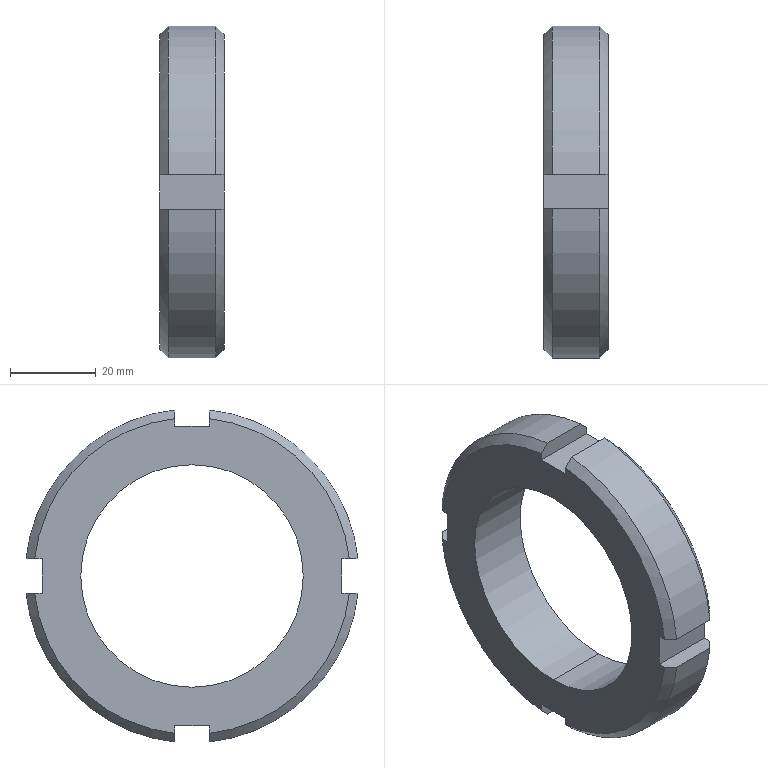Component | SolidWorks | 4RoundNutM52X1.5-1 | 1 solid | 28 faces | box 15 x 77.59 x 77.59 mm | volume 37097 mm3 | plane 14 | cone 8 | cylinder 6 | commonest cylinder face diameters 78 x4 52 x2
build123d program:
from build123d import *

# Parameters (mm, degrees)
SKETCH1_R              = 39
BOSS_EXTRUDE1_DEPTH    = 15
M52X5_0_TAPPED_HOLE1_D = 52
SKETCH5_W              = 8
SKETCH5_H              = 8
CUT_EXTRUDE1_DEPTH     = 15
CIRPATTERN1_COUNT      = 4
CHAMFER1_SIZE          = 2


with BuildPart() as part:
    # Sketch1 → Boss-Extrude1 (new body)
    with BuildSketch(Plane.XY):
        Circle(SKETCH1_R)
    extrude(amount=BOSS_EXTRUDE1_DEPTH)

    # M52x5.0 Tapped Hole1 (through all)
    with Locations(Plane.XY.offset(15)):
        with Locations((0, 0)):
            Hole(M52X5_0_TAPPED_HOLE1_D / 2)

    # Sketch5 → Cut-Extrude1 (cut)
    with BuildSketch(Plane.XY.offset(15)):
        with Locations((0, 39)):
            Rectangle(SKETCH5_W, SKETCH5_H)
    cut_extrude1 = extrude(amount=-CUT_EXTRUDE1_DEPTH, mode=Mode.SUBTRACT)

    # CirPattern1: Cut-Extrude1 ×4 about axis
    cirpattern1_axis = Axis((0, 0, 0), (0, 0, 1))
    for i in range(1, CIRPATTERN1_COUNT):
        add(cut_extrude1.rotate(cirpattern1_axis, i * 360 / CIRPATTERN1_COUNT), mode=Mode.SUBTRACT)

    # Chamfer1
    chamfer1_edges = [part.edges().sort_by_distance(p)[0] for p in [
        (-27.577, 27.577, 0),
        (-27.577, 27.577, 15),
        (27.577, 27.577, 0),
        (27.577, 27.577, 15),
        (-27.577, -27.577, 0),
        (27.577, -27.577, 0),
        (-27.577, -27.577, 15),
        (27.577, -27.577, 15),
    ]]
    chamfer(chamfer1_edges, length=CHAMFER1_SIZE)


solid = part.part

# Placed as in the assembly
solid = solid.moved(Location((72.957, 1.776, 250), (0, 90, 0)))
STEP:
#1=COLOUR_RGB('',0.7922,0.8196,0.9333);
#2=FILL_AREA_STYLE_COLOUR('',#1);
#3=FILL_AREA_STYLE('',(#2));
#4=SURFACE_STYLE_FILL_AREA(#3);
#5=SURFACE_SIDE_STYLE('',(#4));
#6=SURFACE_STYLE_USAGE(.BOTH.,#5);
#7=PRESENTATION_STYLE_ASSIGNMENT((#6));
#8=CARTESIAN_POINT('',(3.463,0.06992,8.819));
#9=VERTEX_POINT('',#8);
#10=CARTESIAN_POINT('',(3.463,0.06992,10.866));
#11=VERTEX_POINT('',#10);
#12=CARTESIAN_POINT('',(3.463,0.06992,9.843));
#13=DIRECTION('',(-1.,-0.,-0.));
#14=DIRECTION('',(0.,0.,1.));
#15=AXIS2_PLACEMENT_3D('',#12,#13,#14);
#16=CIRCLE('',#15,1.024);
#17=EDGE_CURVE('',#9,#11,#16,.T.);
#18=ORIENTED_EDGE('',*,*,#17,.F.);
#19=CARTESIAN_POINT('',(2.872,0.06992,8.819));
#20=VERTEX_POINT('',#19);
#21=CARTESIAN_POINT('',(2.872,0.06992,8.819));
#22=DIRECTION('',(-1.,-0.,-0.));
#23=VECTOR('',#22,39.37);
#24=LINE('',#21,#23);
#25=EDGE_CURVE('',#9,#20,#24,.T.);
#26=ORIENTED_EDGE('',*,*,#25,.T.);
#27=CARTESIAN_POINT('',(2.872,0.06992,10.866));
#28=VERTEX_POINT('',#27);
#29=CARTESIAN_POINT('',(2.872,0.06992,9.843));
#30=DIRECTION('',(-1.,-0.,-0.));
#31=DIRECTION('',(0.,0.,1.));
#32=AXIS2_PLACEMENT_3D('',#29,#30,#31);
#33=CIRCLE('',#32,1.024);
#34=EDGE_CURVE('',#20,#28,#33,.T.);
#35=ORIENTED_EDGE('',*,*,#34,.T.);
#36=CARTESIAN_POINT('',(2.872,0.06992,10.866));
#37=DIRECTION('',(-1.,-0.,-0.));
#38=VECTOR('',#37,39.37);
#39=LINE('',#36,#38);
#40=EDGE_CURVE('',#11,#28,#39,.T.);
#41=ORIENTED_EDGE('',*,*,#40,.F.);
#42=EDGE_LOOP('',(#18,#26,#35,#41));
#43=FACE_OUTER_BOUND('',#42,.T.);
#44=CARTESIAN_POINT('',(2.872,0.06992,9.843));
#45=DIRECTION('',(-1.,-0.,-0.));
#46=DIRECTION('',(0.,0.,1.));
#47=AXIS2_PLACEMENT_3D('',#44,#45,#46);
#48=CYLINDRICAL_SURFACE('',#47,1.024);
#49=ADVANCED_FACE('',(#43),#48,.F.);
#50=CARTESIAN_POINT('',(2.951,-0.08756,8.315));
#51=VERTEX_POINT('',#50);
#52=CARTESIAN_POINT('',(3.384,-0.08756,8.315));
#53=VERTEX_POINT('',#52);
#54=CARTESIAN_POINT('',(2.872,-0.08756,8.315));
#55=DIRECTION('',(1.,0.,0.));
#56=VECTOR('',#55,39.37);
#57=LINE('',#54,#56);
#58=EDGE_CURVE('',#51,#53,#57,.T.);
#59=ORIENTED_EDGE('',*,*,#58,.T.);
#60=CARTESIAN_POINT('',(3.384,-1.457,9.685));
#61=VERTEX_POINT('',#60);
#62=CARTESIAN_POINT('',(3.384,0.06992,9.843));
#63=DIRECTION('',(-1.,-0.,-0.));
#64=DIRECTION('',(0.,-0.,1.));
#65=AXIS2_PLACEMENT_3D('',#62,#63,#64);
#66=CIRCLE('',#65,1.535);
#67=EDGE_CURVE('',#53,#61,#66,.T.);
#68=ORIENTED_EDGE('',*,*,#67,.T.);
#69=CARTESIAN_POINT('',(2.951,-1.457,9.685));
#70=VERTEX_POINT('',#69);
#71=CARTESIAN_POINT('',(2.872,-1.457,9.685));
#72=DIRECTION('',(-1.,-0.,-0.));
#73=VECTOR('',#72,39.37);
#74=LINE('',#71,#73);
#75=EDGE_CURVE('',#61,#70,#74,.T.);
#76=ORIENTED_EDGE('',*,*,#75,.T.);
#77=CARTESIAN_POINT('',(2.951,0.06992,9.843));
#78=DIRECTION('',(1.,0.,0.));
#79=DIRECTION('',(0.,-0.,1.));
#80=AXIS2_PLACEMENT_3D('',#77,#78,#79);
#81=CIRCLE('',#80,1.535);
#82=EDGE_CURVE('',#70,#51,#81,.T.);
#83=ORIENTED_EDGE('',*,*,#82,.T.);
#84=EDGE_LOOP('',(#59,#68,#76,#83));
#85=FACE_OUTER_BOUND('',#84,.T.);
#86=CARTESIAN_POINT('',(2.872,0.06992,9.843));
#87=DIRECTION('',(1.,0.,0.));
#88=DIRECTION('',(0.,0.,-1.));
#89=AXIS2_PLACEMENT_3D('',#86,#87,#88);
#90=CYLINDRICAL_SURFACE('',#89,1.535);
#91=ADVANCED_FACE('',(#85),#90,.T.);
#92=CARTESIAN_POINT('',(2.951,1.597,9.685));
#93=VERTEX_POINT('',#92);
#94=CARTESIAN_POINT('',(3.384,1.597,9.685));
#95=VERTEX_POINT('',#94);
#96=CARTESIAN_POINT('',(2.872,1.597,9.685));
#97=DIRECTION('',(1.,0.,0.));
#98=VECTOR('',#97,39.37);
#99=LINE('',#96,#98);
#100=EDGE_CURVE('',#93,#95,#99,.T.);
#101=ORIENTED_EDGE('',*,*,#100,.T.);
#102=CARTESIAN_POINT('',(3.384,0.2274,8.315));
#103=VERTEX_POINT('',#102);
#104=CARTESIAN_POINT('',(3.384,0.06992,9.843));
#105=DIRECTION('',(-1.,-0.,-0.));
#106=DIRECTION('',(0.,-0.,1.));
#107=AXIS2_PLACEMENT_3D('',#104,#105,#106);
#108=CIRCLE('',#107,1.535);
#109=EDGE_CURVE('',#95,#103,#108,.T.);
#110=ORIENTED_EDGE('',*,*,#109,.T.);
#111=CARTESIAN_POINT('',(2.951,0.2274,8.315));
#112=VERTEX_POINT('',#111);
#113=CARTESIAN_POINT('',(2.872,0.2274,8.315));
#114=DIRECTION('',(-1.,-0.,-0.));
#115=VECTOR('',#114,39.37);
#116=LINE('',#113,#115);
#117=EDGE_CURVE('',#103,#112,#116,.T.);
#118=ORIENTED_EDGE('',*,*,#117,.T.);
#119=CARTESIAN_POINT('',(2.951,0.06992,9.843));
#120=DIRECTION('',(1.,0.,0.));
#121=DIRECTION('',(0.,-0.,1.));
#122=AXIS2_PLACEMENT_3D('',#119,#120,#121);
#123=CIRCLE('',#122,1.535);
#124=EDGE_CURVE('',#112,#93,#123,.T.);
#125=ORIENTED_EDGE('',*,*,#124,.T.);
#126=EDGE_LOOP('',(#101,#110,#118,#125));
#127=FACE_OUTER_BOUND('',#126,.T.);
#128=CARTESIAN_POINT('',(2.872,0.06992,9.843));
#129=DIRECTION('',(1.,0.,0.));
#130=DIRECTION('',(0.,0.,-1.));
#131=AXIS2_PLACEMENT_3D('',#128,#129,#130);
#132=CYLINDRICAL_SURFACE('',#131,1.535);
#133=ADVANCED_FACE('',(#127),#132,.T.);
#134=CARTESIAN_POINT('',(2.951,-1.457,10.));
#135=VERTEX_POINT('',#134);
#136=CARTESIAN_POINT('',(3.384,-1.457,10.));
#137=VERTEX_POINT('',#136);
#138=CARTESIAN_POINT('',(2.872,-1.457,10.));
#139=DIRECTION('',(1.,0.,0.));
#140=VECTOR('',#139,39.37);
#141=LINE('',#138,#140);
#142=EDGE_CURVE('',#135,#137,#141,.T.);
#143=ORIENTED_EDGE('',*,*,#142,.T.);
#144=CARTESIAN_POINT('',(3.384,-0.08756,11.37));
#145=VERTEX_POINT('',#144);
#146=CARTESIAN_POINT('',(3.384,0.06992,9.843));
#147=DIRECTION('',(-1.,-0.,-0.));
#148=DIRECTION('',(0.,-0.,1.));
#149=AXIS2_PLACEMENT_3D('',#146,#147,#148);
#150=CIRCLE('',#149,1.535);
#151=EDGE_CURVE('',#137,#145,#150,.T.);
#152=ORIENTED_EDGE('',*,*,#151,.T.);
#153=CARTESIAN_POINT('',(2.951,-0.08756,11.37));
#154=VERTEX_POINT('',#153);
#155=CARTESIAN_POINT('',(2.872,-0.08756,11.37));
#156=DIRECTION('',(-1.,-0.,-0.));
#157=VECTOR('',#156,39.37);
#158=LINE('',#155,#157);
#159=EDGE_CURVE('',#145,#154,#158,.T.);
#160=ORIENTED_EDGE('',*,*,#159,.T.);
#161=CARTESIAN_POINT('',(2.951,0.06992,9.843));
#162=DIRECTION('',(1.,0.,0.));
#163=DIRECTION('',(0.,-0.,1.));
#164=AXIS2_PLACEMENT_3D('',#161,#162,#163);
#165=CIRCLE('',#164,1.535);
#166=EDGE_CURVE('',#154,#135,#165,.T.);
#167=ORIENTED_EDGE('',*,*,#166,.T.);
#168=EDGE_LOOP('',(#143,#152,#160,#167));
#169=FACE_OUTER_BOUND('',#168,.T.);
#170=CARTESIAN_POINT('',(2.872,0.06992,9.843));
#171=DIRECTION('',(1.,0.,0.));
#172=DIRECTION('',(0.,0.,-1.));
#173=AXIS2_PLACEMENT_3D('',#170,#171,#172);
#174=CYLINDRICAL_SURFACE('',#173,1.535);
#175=ADVANCED_FACE('',(#169),#174,.T.);
#176=CARTESIAN_POINT('',(2.951,0.2274,11.37));
#177=VERTEX_POINT('',#176);
#178=CARTESIAN_POINT('',(3.384,0.2274,11.37));
#179=VERTEX_POINT('',#178);
#180=CARTESIAN_POINT('',(2.872,0.2274,11.37));
#181=DIRECTION('',(1.,0.,0.));
#182=VECTOR('',#181,39.37);
#183=LINE('',#180,#182);
#184=EDGE_CURVE('',#177,#179,#183,.T.);
#185=ORIENTED_EDGE('',*,*,#184,.T.);
#186=CARTESIAN_POINT('',(3.384,1.597,10.));
#187=VERTEX_POINT('',#186);
#188=CARTESIAN_POINT('',(3.384,0.06992,9.843));
#189=DIRECTION('',(-1.,-0.,-0.));
#190=DIRECTION('',(0.,-0.,1.));
#191=AXIS2_PLACEMENT_3D('',#188,#189,#190);
#192=CIRCLE('',#191,1.535);
#193=EDGE_CURVE('',#179,#187,#192,.T.);
#194=ORIENTED_EDGE('',*,*,#193,.T.);
#195=CARTESIAN_POINT('',(2.951,1.597,10.));
#196=VERTEX_POINT('',#195);
#197=CARTESIAN_POINT('',(2.872,1.597,10.));
#198=DIRECTION('',(-1.,-0.,-0.));
#199=VECTOR('',#198,39.37);
#200=LINE('',#197,#199);
#201=EDGE_CURVE('',#187,#196,#200,.T.);
#202=ORIENTED_EDGE('',*,*,#201,.T.);
#203=CARTESIAN_POINT('',(2.951,0.06992,9.843));
#204=DIRECTION('',(1.,0.,0.));
#205=DIRECTION('',(0.,-0.,1.));
#206=AXIS2_PLACEMENT_3D('',#203,#204,#205);
#207=CIRCLE('',#206,1.535);
#208=EDGE_CURVE('',#196,#177,#207,.T.);
#209=ORIENTED_EDGE('',*,*,#208,.T.);
#210=EDGE_LOOP('',(#185,#194,#202,#209));
#211=FACE_OUTER_BOUND('',#210,.T.);
#212=CARTESIAN_POINT('',(2.872,0.06992,9.843));
#213=DIRECTION('',(1.,0.,0.));
#214=DIRECTION('',(0.,0.,-1.));
#215=AXIS2_PLACEMENT_3D('',#212,#213,#214);
#216=CYLINDRICAL_SURFACE('',#215,1.535);
#217=ADVANCED_FACE('',(#211),#216,.T.);
#218=CARTESIAN_POINT('',(2.872,-1.378,10.));
#219=VERTEX_POINT('',#218);
#220=CARTESIAN_POINT('',(2.872,-1.308,10.));
#221=VERTEX_POINT('',#220);
#222=CARTESIAN_POINT('',(2.872,-1.308,10.));
#223=DIRECTION('',(-0.,1.,0.));
#224=VECTOR('',#223,39.37);
#225=LINE('',#222,#224);
#226=EDGE_CURVE('',#219,#221,#225,.T.);
#227=ORIENTED_EDGE('',*,*,#226,.F.);
#228=CARTESIAN_POINT('',(2.872,-0.08756,11.291));
#229=VERTEX_POINT('',#228);
#230=CARTESIAN_POINT('',(2.872,0.06992,9.843));
#231=DIRECTION('',(-1.,-0.,-0.));
#232=DIRECTION('',(0.,-0.,1.));
#233=AXIS2_PLACEMENT_3D('',#230,#231,#232);
#234=CIRCLE('',#233,1.457);
#235=EDGE_CURVE('',#219,#229,#234,.T.);
#236=ORIENTED_EDGE('',*,*,#235,.T.);
#237=CARTESIAN_POINT('',(2.872,-0.08756,11.22));
#238=VERTEX_POINT('',#237);
#239=CARTESIAN_POINT('',(2.872,-0.08756,11.22));
#240=DIRECTION('',(-0.,-0.,1.));
#241=VECTOR('',#240,39.37);
#242=LINE('',#239,#241);
#243=EDGE_CURVE('',#238,#229,#242,.T.);
#244=ORIENTED_EDGE('',*,*,#243,.F.);
#245=CARTESIAN_POINT('',(2.872,0.2274,11.22));
#246=VERTEX_POINT('',#245);
#247=CARTESIAN_POINT('',(2.872,0.2274,11.22));
#248=DIRECTION('',(0.,-1.,-0.));
#249=VECTOR('',#248,39.37);
#250=LINE('',#247,#249);
#251=EDGE_CURVE('',#246,#238,#250,.T.);
#252=ORIENTED_EDGE('',*,*,#251,.F.);
#253=CARTESIAN_POINT('',(2.872,0.2274,11.291));
#254=VERTEX_POINT('',#253);
#255=CARTESIAN_POINT('',(2.872,0.2274,11.22));
#256=DIRECTION('',(0.,0.,-1.));
#257=VECTOR('',#256,39.37);
#258=LINE('',#255,#257);
#259=EDGE_CURVE('',#254,#246,#258,.T.);
#260=ORIENTED_EDGE('',*,*,#259,.F.);
#261=CARTESIAN_POINT('',(2.872,1.518,10.));
#262=VERTEX_POINT('',#261);
#263=CARTESIAN_POINT('',(2.872,0.06992,9.843));
#264=DIRECTION('',(-1.,-0.,-0.));
#265=DIRECTION('',(0.,-0.,1.));
#266=AXIS2_PLACEMENT_3D('',#263,#264,#265);
#267=CIRCLE('',#266,1.457);
#268=EDGE_CURVE('',#254,#262,#267,.T.);
#269=ORIENTED_EDGE('',*,*,#268,.T.);
#270=CARTESIAN_POINT('',(2.872,1.448,10.));
#271=VERTEX_POINT('',#270);
#272=CARTESIAN_POINT('',(2.872,1.448,10.));
#273=DIRECTION('',(-0.,1.,0.));
#274=VECTOR('',#273,39.37);
#275=LINE('',#272,#274);
#276=EDGE_CURVE('',#271,#262,#275,.T.);
#277=ORIENTED_EDGE('',*,*,#276,.F.);
#278=CARTESIAN_POINT('',(2.872,1.448,9.685));
#279=VERTEX_POINT('',#278);
#280=CARTESIAN_POINT('',(2.872,1.448,9.685));
#281=DIRECTION('',(-0.,-0.,1.));
#282=VECTOR('',#281,39.37);
#283=LINE('',#280,#282);
#284=EDGE_CURVE('',#279,#271,#283,.T.);
#285=ORIENTED_EDGE('',*,*,#284,.F.);
#286=CARTESIAN_POINT('',(2.872,1.518,9.685));
#287=VERTEX_POINT('',#286);
#288=CARTESIAN_POINT('',(2.872,1.448,9.685));
#289=DIRECTION('',(0.,-1.,-0.));
#290=VECTOR('',#289,39.37);
#291=LINE('',#288,#290);
#292=EDGE_CURVE('',#287,#279,#291,.T.);
#293=ORIENTED_EDGE('',*,*,#292,.F.);
#294=CARTESIAN_POINT('',(2.872,0.2274,8.394));
#295=VERTEX_POINT('',#294);
#296=CARTESIAN_POINT('',(2.872,0.06992,9.843));
#297=DIRECTION('',(-1.,-0.,-0.));
#298=DIRECTION('',(0.,-0.,1.));
#299=AXIS2_PLACEMENT_3D('',#296,#297,#298);
#300=CIRCLE('',#299,1.457);
#301=EDGE_CURVE('',#287,#295,#300,.T.);
#302=ORIENTED_EDGE('',*,*,#301,.T.);
#303=CARTESIAN_POINT('',(2.872,0.2274,8.465));
#304=VERTEX_POINT('',#303);
#305=CARTESIAN_POINT('',(2.872,0.2274,8.465));
#306=DIRECTION('',(0.,0.,-1.));
#307=VECTOR('',#306,39.37);
#308=LINE('',#305,#307);
#309=EDGE_CURVE('',#304,#295,#308,.T.);
#310=ORIENTED_EDGE('',*,*,#309,.F.);
#311=CARTESIAN_POINT('',(2.872,-0.08756,8.465));
#312=VERTEX_POINT('',#311);
#313=CARTESIAN_POINT('',(2.872,-0.08756,8.465));
#314=DIRECTION('',(-0.,1.,0.));
#315=VECTOR('',#314,39.37);
#316=LINE('',#313,#315);
#317=EDGE_CURVE('',#312,#304,#316,.T.);
#318=ORIENTED_EDGE('',*,*,#317,.F.);
#319=CARTESIAN_POINT('',(2.872,-0.08756,8.394));
#320=VERTEX_POINT('',#319);
#321=CARTESIAN_POINT('',(2.872,-0.08756,8.465));
#322=DIRECTION('',(-0.,-0.,1.));
#323=VECTOR('',#322,39.37);
#324=LINE('',#321,#323);
#325=EDGE_CURVE('',#320,#312,#324,.T.);
#326=ORIENTED_EDGE('',*,*,#325,.F.);
#327=CARTESIAN_POINT('',(2.872,-1.378,9.685));
#328=VERTEX_POINT('',#327);
#329=CARTESIAN_POINT('',(2.872,0.06992,9.843));
#330=DIRECTION('',(-1.,-0.,-0.));
#331=DIRECTION('',(0.,-0.,1.));
#332=AXIS2_PLACEMENT_3D('',#329,#330,#331);
#333=CIRCLE('',#332,1.457);
#334=EDGE_CURVE('',#320,#328,#333,.T.);
#335=ORIENTED_EDGE('',*,*,#334,.T.);
#336=CARTESIAN_POINT('',(2.872,-1.308,9.685));
#337=VERTEX_POINT('',#336);
#338=CARTESIAN_POINT('',(2.872,-1.308,9.685));
#339=DIRECTION('',(0.,-1.,-0.));
#340=VECTOR('',#339,39.37);
#341=LINE('',#338,#340);
#342=EDGE_CURVE('',#337,#328,#341,.T.);
#343=ORIENTED_EDGE('',*,*,#342,.F.);
#344=CARTESIAN_POINT('',(2.872,-1.308,10.));
#345=DIRECTION('',(0.,0.,-1.));
#346=VECTOR('',#345,39.37);
#347=LINE('',#344,#346);
#348=EDGE_CURVE('',#221,#337,#347,.T.);
#349=ORIENTED_EDGE('',*,*,#348,.F.);
#350=EDGE_LOOP('',(#227,#236,#244,#252,#260,#269,#277,#285,#293,#302,#310,#318,#326,#335,#343,#349));
#351=FACE_OUTER_BOUND('',#350,.T.);
#352=CARTESIAN_POINT('',(2.872,0.06992,9.843));
#353=DIRECTION('',(-1.,-0.,-0.));
#354=DIRECTION('',(0.,0.,1.));
#355=AXIS2_PLACEMENT_3D('',#352,#353,#354);
#356=CIRCLE('',#355,1.024);
#357=EDGE_CURVE('',#28,#20,#356,.T.);
#358=ORIENTED_EDGE('',*,*,#357,.F.);
#359=ORIENTED_EDGE('',*,*,#34,.F.);
#360=EDGE_LOOP('',(#358,#359));
#361=FACE_BOUND('',#360,.T.);
#362=CARTESIAN_POINT('',(2.872,0.06992,9.843));
#363=DIRECTION('',(-1.,-0.,-0.));
#364=DIRECTION('',(-0.,-0.,1.));
#365=AXIS2_PLACEMENT_3D('',#362,#363,#364);
#366=PLANE('',#365);
#367=ADVANCED_FACE('',(#351,#361),#366,.T.);
#368=CARTESIAN_POINT('',(3.463,0.06992,9.843));
#369=DIRECTION('',(-1.,-0.,-0.));
#370=DIRECTION('',(0.,0.,1.));
#371=AXIS2_PLACEMENT_3D('',#368,#369,#370);
#372=CIRCLE('',#371,1.024);
#373=EDGE_CURVE('',#11,#9,#372,.T.);
#374=ORIENTED_EDGE('',*,*,#373,.T.);
#375=ORIENTED_EDGE('',*,*,#17,.T.);
#376=EDGE_LOOP('',(#374,#375));
#377=FACE_BOUND('',#376,.T.);
#378=CARTESIAN_POINT('',(3.463,0.2274,8.465));
#379=VERTEX_POINT('',#378);
#380=CARTESIAN_POINT('',(3.463,0.2274,8.394));
#381=VERTEX_POINT('',#380);
#382=CARTESIAN_POINT('',(3.463,0.2274,8.465));
#383=DIRECTION('',(0.,0.,-1.));
#384=VECTOR('',#383,39.37);
#385=LINE('',#382,#384);
#386=EDGE_CURVE('',#379,#381,#385,.T.);
#387=ORIENTED_EDGE('',*,*,#386,.T.);
#388=CARTESIAN_POINT('',(3.463,1.518,9.685));
#389=VERTEX_POINT('',#388);
#390=CARTESIAN_POINT('',(3.463,0.06992,9.843));
#391=DIRECTION('',(1.,0.,0.));
#392=DIRECTION('',(0.,-0.,1.));
#393=AXIS2_PLACEMENT_3D('',#390,#391,#392);
#394=CIRCLE('',#393,1.457);
#395=EDGE_CURVE('',#381,#389,#394,.T.);
#396=ORIENTED_EDGE('',*,*,#395,.T.);
#397=CARTESIAN_POINT('',(3.463,1.448,9.685));
#398=VERTEX_POINT('',#397);
#399=CARTESIAN_POINT('',(3.463,0.06992,9.685));
#400=DIRECTION('',(0.,-1.,-0.));
#401=VECTOR('',#400,39.37);
#402=LINE('',#399,#401);
#403=EDGE_CURVE('',#389,#398,#402,.T.);
#404=ORIENTED_EDGE('',*,*,#403,.T.);
#405=CARTESIAN_POINT('',(3.463,1.448,10.));
#406=VERTEX_POINT('',#405);
#407=CARTESIAN_POINT('',(3.463,1.448,9.685));
#408=DIRECTION('',(-0.,-0.,1.));
#409=VECTOR('',#408,39.37);
#410=LINE('',#407,#409);
#411=EDGE_CURVE('',#398,#406,#410,.T.);
#412=ORIENTED_EDGE('',*,*,#411,.T.);
#413=CARTESIAN_POINT('',(3.463,1.518,10.));
#414=VERTEX_POINT('',#413);
#415=CARTESIAN_POINT('',(3.463,1.448,10.));
#416=DIRECTION('',(-0.,1.,0.));
#417=VECTOR('',#416,39.37);
#418=LINE('',#415,#417);
#419=EDGE_CURVE('',#406,#414,#418,.T.);
#420=ORIENTED_EDGE('',*,*,#419,.T.);
#421=CARTESIAN_POINT('',(3.463,0.2274,11.291));
#422=VERTEX_POINT('',#421);
#423=CARTESIAN_POINT('',(3.463,0.06992,9.843));
#424=DIRECTION('',(1.,0.,0.));
#425=DIRECTION('',(0.,-0.,1.));
#426=AXIS2_PLACEMENT_3D('',#423,#424,#425);
#427=CIRCLE('',#426,1.457);
#428=EDGE_CURVE('',#414,#422,#427,.T.);
#429=ORIENTED_EDGE('',*,*,#428,.T.);
#430=CARTESIAN_POINT('',(3.463,0.2274,11.22));
#431=VERTEX_POINT('',#430);
#432=CARTESIAN_POINT('',(3.463,0.2274,9.843));
#433=DIRECTION('',(0.,0.,-1.));
#434=VECTOR('',#433,39.37);
#435=LINE('',#432,#434);
#436=EDGE_CURVE('',#422,#431,#435,.T.);
#437=ORIENTED_EDGE('',*,*,#436,.T.);
#438=CARTESIAN_POINT('',(3.463,-0.08756,11.22));
#439=VERTEX_POINT('',#438);
#440=CARTESIAN_POINT('',(3.463,0.2274,11.22));
#441=DIRECTION('',(0.,-1.,-0.));
#442=VECTOR('',#441,39.37);
#443=LINE('',#440,#442);
#444=EDGE_CURVE('',#431,#439,#443,.T.);
#445=ORIENTED_EDGE('',*,*,#444,.T.);
#446=CARTESIAN_POINT('',(3.463,-0.08756,11.291));
#447=VERTEX_POINT('',#446);
#448=CARTESIAN_POINT('',(3.463,-0.08756,11.22));
#449=DIRECTION('',(-0.,-0.,1.));
#450=VECTOR('',#449,39.37);
#451=LINE('',#448,#450);
#452=EDGE_CURVE('',#439,#447,#451,.T.);
#453=ORIENTED_EDGE('',*,*,#452,.T.);
#454=CARTESIAN_POINT('',(3.463,-1.378,10.));
#455=VERTEX_POINT('',#454);
#456=CARTESIAN_POINT('',(3.463,0.06992,9.843));
#457=DIRECTION('',(1.,0.,0.));
#458=DIRECTION('',(0.,-0.,1.));
#459=AXIS2_PLACEMENT_3D('',#456,#457,#458);
#460=CIRCLE('',#459,1.457);
#461=EDGE_CURVE('',#447,#455,#460,.T.);
#462=ORIENTED_EDGE('',*,*,#461,.T.);
#463=CARTESIAN_POINT('',(3.463,-1.308,10.));
#464=VERTEX_POINT('',#463);
#465=CARTESIAN_POINT('',(3.463,0.06992,10.));
#466=DIRECTION('',(-0.,1.,0.));
#467=VECTOR('',#466,39.37);
#468=LINE('',#465,#467);
#469=EDGE_CURVE('',#455,#464,#468,.T.);
#470=ORIENTED_EDGE('',*,*,#469,.T.);
#471=CARTESIAN_POINT('',(3.463,-1.308,9.685));
#472=VERTEX_POINT('',#471);
#473=CARTESIAN_POINT('',(3.463,-1.308,10.));
#474=DIRECTION('',(0.,0.,-1.));
#475=VECTOR('',#474,39.37);
#476=LINE('',#473,#475);
#477=EDGE_CURVE('',#464,#472,#476,.T.);
#478=ORIENTED_EDGE('',*,*,#477,.T.);
#479=CARTESIAN_POINT('',(3.463,-1.378,9.685));
#480=VERTEX_POINT('',#479);
#481=CARTESIAN_POINT('',(3.463,-1.308,9.685));
#482=DIRECTION('',(0.,-1.,-0.));
#483=VECTOR('',#482,39.37);
#484=LINE('',#481,#483);
#485=EDGE_CURVE('',#472,#480,#484,.T.);
#486=ORIENTED_EDGE('',*,*,#485,.T.);
#487=CARTESIAN_POINT('',(3.463,-0.08756,8.394));
#488=VERTEX_POINT('',#487);
#489=CARTESIAN_POINT('',(3.463,0.06992,9.843));
#490=DIRECTION('',(1.,0.,0.));
#491=DIRECTION('',(0.,-0.,1.));
#492=AXIS2_PLACEMENT_3D('',#489,#490,#491);
#493=CIRCLE('',#492,1.457);
#494=EDGE_CURVE('',#480,#488,#493,.T.);
#495=ORIENTED_EDGE('',*,*,#494,.T.);
#496=CARTESIAN_POINT('',(3.463,-0.08756,8.465));
#497=VERTEX_POINT('',#496);
#498=CARTESIAN_POINT('',(3.463,-0.08756,9.843));
#499=DIRECTION('',(-0.,-0.,1.));
#500=VECTOR('',#499,39.37);
#501=LINE('',#498,#500);
#502=EDGE_CURVE('',#488,#497,#501,.T.);
#503=ORIENTED_EDGE('',*,*,#502,.T.);
#504=CARTESIAN_POINT('',(3.463,-0.08756,8.465));
#505=DIRECTION('',(-0.,1.,0.));
#506=VECTOR('',#505,39.37);
#507=LINE('',#504,#506);
#508=EDGE_CURVE('',#497,#379,#507,.T.);
#509=ORIENTED_EDGE('',*,*,#508,.T.);
#510=EDGE_LOOP('',(#387,#396,#404,#412,#420,#429,#437,#445,#453,#462,#470,#478,#486,#495,#503,#509));
#511=FACE_OUTER_BOUND('',#510,.T.);
#512=CARTESIAN_POINT('',(3.463,0.06992,9.843));
#513=DIRECTION('',(-1.,-0.,-0.));
#514=DIRECTION('',(-0.,-0.,1.));
#515=AXIS2_PLACEMENT_3D('',#512,#513,#514);
#516=PLANE('',#515);
#517=ADVANCED_FACE('',(#377,#511),#516,.F.);
#518=ORIENTED_EDGE('',*,*,#25,.F.);
#519=ORIENTED_EDGE('',*,*,#373,.F.);
#520=ORIENTED_EDGE('',*,*,#40,.T.);
#521=ORIENTED_EDGE('',*,*,#357,.T.);
#522=EDGE_LOOP('',(#518,#519,#520,#521));
#523=FACE_OUTER_BOUND('',#522,.T.);
#524=CARTESIAN_POINT('',(2.872,0.06992,9.843));
#525=DIRECTION('',(-1.,-0.,-0.));
#526=DIRECTION('',(0.,0.,1.));
#527=AXIS2_PLACEMENT_3D('',#524,#525,#526);
#528=CYLINDRICAL_SURFACE('',#527,1.024);
#529=ADVANCED_FACE('',(#523),#528,.F.);
#530=ORIENTED_EDGE('',*,*,#201,.F.);
#531=CARTESIAN_POINT('',(3.384,1.597,10.));
#532=CARTESIAN_POINT('',(3.41,1.571,10.));
#533=CARTESIAN_POINT('',(3.437,1.544,10.));
#534=CARTESIAN_POINT('',(3.463,1.518,10.));
#535=B_SPLINE_CURVE_WITH_KNOTS('',3,(#531,#532,#533,#534),.UNSPECIFIED.,.F.,.F.,(4,4),(0.,0.002836),.UNSPECIFIED.);
#536=EDGE_CURVE('',#187,#414,#535,.T.);
#537=ORIENTED_EDGE('',*,*,#536,.T.);
#538=ORIENTED_EDGE('',*,*,#419,.F.);
#539=CARTESIAN_POINT('',(3.463,1.448,10.));
#540=DIRECTION('',(-1.,-0.,-0.));
#541=VECTOR('',#540,39.37);
#542=LINE('',#539,#541);
#543=EDGE_CURVE('',#406,#271,#542,.T.);
#544=ORIENTED_EDGE('',*,*,#543,.T.);
#545=ORIENTED_EDGE('',*,*,#276,.T.);
#546=CARTESIAN_POINT('',(2.872,1.518,10.));
#547=CARTESIAN_POINT('',(2.899,1.544,10.));
#548=CARTESIAN_POINT('',(2.925,1.571,10.));
#549=CARTESIAN_POINT('',(2.951,1.597,10.));
#550=B_SPLINE_CURVE_WITH_KNOTS('',3,(#546,#547,#548,#549),.UNSPECIFIED.,.F.,.F.,(4,4),(0.,0.002836),.UNSPECIFIED.);
#551=EDGE_CURVE('',#262,#196,#550,.T.);
#552=ORIENTED_EDGE('',*,*,#551,.T.);
#553=EDGE_LOOP('',(#530,#537,#538,#544,#545,#552));
#554=FACE_OUTER_BOUND('',#553,.T.);
#555=CARTESIAN_POINT('',(3.463,1.448,10.));
#556=DIRECTION('',(-0.,-0.,1.));
#557=DIRECTION('',(1.,0.,0.));
#558=AXIS2_PLACEMENT_3D('',#555,#556,#557);
#559=PLANE('',#558);
#560=ADVANCED_FACE('',(#554),#559,.F.);
#561=ORIENTED_EDGE('',*,*,#403,.F.);
#562=CARTESIAN_POINT('',(3.463,1.518,9.685));
#563=CARTESIAN_POINT('',(3.437,1.544,9.685));
#564=CARTESIAN_POINT('',(3.41,1.571,9.685));
#565=CARTESIAN_POINT('',(3.384,1.597,9.685));
#566=B_SPLINE_CURVE_WITH_KNOTS('',3,(#562,#563,#564,#565),.UNSPECIFIED.,.F.,.F.,(4,4),(0.,0.002836),.UNSPECIFIED.);
#567=EDGE_CURVE('',#389,#95,#566,.T.);
#568=ORIENTED_EDGE('',*,*,#567,.T.);
#569=ORIENTED_EDGE('',*,*,#100,.F.);
#570=CARTESIAN_POINT('',(2.951,1.597,9.685));
#571=CARTESIAN_POINT('',(2.925,1.571,9.685));
#572=CARTESIAN_POINT('',(2.899,1.544,9.685));
#573=CARTESIAN_POINT('',(2.872,1.518,9.685));
#574=B_SPLINE_CURVE_WITH_KNOTS('',3,(#570,#571,#572,#573),.UNSPECIFIED.,.F.,.F.,(4,4),(0.,0.002836),.UNSPECIFIED.);
#575=EDGE_CURVE('',#93,#287,#574,.T.);
#576=ORIENTED_EDGE('',*,*,#575,.T.);
#577=ORIENTED_EDGE('',*,*,#292,.T.);
#578=CARTESIAN_POINT('',(3.463,1.448,9.685));
#579=DIRECTION('',(-1.,-0.,-0.));
#580=VECTOR('',#579,39.37);
#581=LINE('',#578,#580);
#582=EDGE_CURVE('',#398,#279,#581,.T.);
#583=ORIENTED_EDGE('',*,*,#582,.F.);
#584=EDGE_LOOP('',(#561,#568,#569,#576,#577,#583));
#585=FACE_OUTER_BOUND('',#584,.T.);
#586=CARTESIAN_POINT('',(3.463,1.448,9.685));
#587=DIRECTION('',(0.,0.,-1.));
#588=DIRECTION('',(-1.,-0.,-0.));
#589=AXIS2_PLACEMENT_3D('',#586,#587,#588);
#590=PLANE('',#589);
#591=ADVANCED_FACE('',(#585),#590,.F.);
#592=ORIENTED_EDGE('',*,*,#284,.T.);
#593=ORIENTED_EDGE('',*,*,#543,.F.);
#594=ORIENTED_EDGE('',*,*,#411,.F.);
#595=ORIENTED_EDGE('',*,*,#582,.T.);
#596=EDGE_LOOP('',(#592,#593,#594,#595));
#597=FACE_OUTER_BOUND('',#596,.T.);
#598=CARTESIAN_POINT('',(3.463,1.448,9.685));
#599=DIRECTION('',(0.,-1.,-0.));
#600=DIRECTION('',(1.,0.,0.));
#601=AXIS2_PLACEMENT_3D('',#598,#599,#600);
#602=PLANE('',#601);
#603=ADVANCED_FACE('',(#597),#602,.F.);
#604=ORIENTED_EDGE('',*,*,#159,.F.);
#605=CARTESIAN_POINT('',(3.384,-0.08756,11.37));
#606=CARTESIAN_POINT('',(3.41,-0.08756,11.343));
#607=CARTESIAN_POINT('',(3.437,-0.08756,11.317));
#608=CARTESIAN_POINT('',(3.463,-0.08756,11.291));
#609=B_SPLINE_CURVE_WITH_KNOTS('',3,(#605,#606,#607,#608),.UNSPECIFIED.,.F.,.F.,(4,4),(0.,0.002836),.UNSPECIFIED.);
#610=EDGE_CURVE('',#145,#447,#609,.T.);
#611=ORIENTED_EDGE('',*,*,#610,.T.);
#612=ORIENTED_EDGE('',*,*,#452,.F.);
#613=CARTESIAN_POINT('',(3.463,-0.08756,11.22));
#614=DIRECTION('',(-1.,-0.,-0.));
#615=VECTOR('',#614,39.37);
#616=LINE('',#613,#615);
#617=EDGE_CURVE('',#439,#238,#616,.T.);
#618=ORIENTED_EDGE('',*,*,#617,.T.);
#619=ORIENTED_EDGE('',*,*,#243,.T.);
#620=CARTESIAN_POINT('',(2.872,-0.08756,11.291));
#621=CARTESIAN_POINT('',(2.899,-0.08756,11.317));
#622=CARTESIAN_POINT('',(2.925,-0.08756,11.343));
#623=CARTESIAN_POINT('',(2.951,-0.08756,11.37));
#624=B_SPLINE_CURVE_WITH_KNOTS('',3,(#620,#621,#622,#623),.UNSPECIFIED.,.F.,.F.,(4,4),(0.,0.002836),.UNSPECIFIED.);
#625=EDGE_CURVE('',#229,#154,#624,.T.);
#626=ORIENTED_EDGE('',*,*,#625,.T.);
#627=EDGE_LOOP('',(#604,#611,#612,#618,#619,#626));
#628=FACE_OUTER_BOUND('',#627,.T.);
#629=CARTESIAN_POINT('',(3.463,-0.08756,11.22));
#630=DIRECTION('',(0.,-1.,-0.));
#631=DIRECTION('',(1.,0.,0.));
#632=AXIS2_PLACEMENT_3D('',#629,#630,#631);
#633=PLANE('',#632);
#634=ADVANCED_FACE('',(#628),#633,.F.);
#635=ORIENTED_EDGE('',*,*,#436,.F.);
#636=CARTESIAN_POINT('',(3.463,0.2274,11.291));
#637=CARTESIAN_POINT('',(3.437,0.2274,11.317));
#638=CARTESIAN_POINT('',(3.41,0.2274,11.343));
#639=CARTESIAN_POINT('',(3.384,0.2274,11.37));
#640=B_SPLINE_CURVE_WITH_KNOTS('',3,(#636,#637,#638,#639),.UNSPECIFIED.,.F.,.F.,(4,4),(0.,0.002836),.UNSPECIFIED.);
#641=EDGE_CURVE('',#422,#179,#640,.T.);
#642=ORIENTED_EDGE('',*,*,#641,.T.);
#643=ORIENTED_EDGE('',*,*,#184,.F.);
#644=CARTESIAN_POINT('',(2.951,0.2274,11.37));
#645=CARTESIAN_POINT('',(2.925,0.2274,11.343));
#646=CARTESIAN_POINT('',(2.899,0.2274,11.317));
#647=CARTESIAN_POINT('',(2.872,0.2274,11.291));
#648=B_SPLINE_CURVE_WITH_KNOTS('',3,(#644,#645,#646,#647),.UNSPECIFIED.,.F.,.F.,(4,4),(0.,0.002836),.UNSPECIFIED.);
#649=EDGE_CURVE('',#177,#254,#648,.T.);
#650=ORIENTED_EDGE('',*,*,#649,.T.);
#651=ORIENTED_EDGE('',*,*,#259,.T.);
#652=CARTESIAN_POINT('',(3.463,0.2274,11.22));
#653=DIRECTION('',(-1.,-0.,-0.));
#654=VECTOR('',#653,39.37);
#655=LINE('',#652,#654);
#656=EDGE_CURVE('',#431,#246,#655,.T.);
#657=ORIENTED_EDGE('',*,*,#656,.F.);
#658=EDGE_LOOP('',(#635,#642,#643,#650,#651,#657));
#659=FACE_OUTER_BOUND('',#658,.T.);
#660=CARTESIAN_POINT('',(3.463,0.2274,11.22));
#661=DIRECTION('',(-0.,1.,0.));
#662=DIRECTION('',(-1.,-0.,-0.));
#663=AXIS2_PLACEMENT_3D('',#660,#661,#662);
#664=PLANE('',#663);
#665=ADVANCED_FACE('',(#659),#664,.F.);
#666=ORIENTED_EDGE('',*,*,#251,.T.);
#667=ORIENTED_EDGE('',*,*,#617,.F.);
#668=ORIENTED_EDGE('',*,*,#444,.F.);
#669=ORIENTED_EDGE('',*,*,#656,.T.);
#670=EDGE_LOOP('',(#666,#667,#668,#669));
#671=FACE_OUTER_BOUND('',#670,.T.);
#672=CARTESIAN_POINT('',(3.463,0.2274,11.22));
#673=DIRECTION('',(0.,0.,-1.));
#674=DIRECTION('',(1.,0.,0.));
#675=AXIS2_PLACEMENT_3D('',#672,#673,#674);
#676=PLANE('',#675);
#677=ADVANCED_FACE('',(#671),#676,.F.);
#678=ORIENTED_EDGE('',*,*,#117,.F.);
#679=CARTESIAN_POINT('',(3.384,0.2274,8.315));
#680=CARTESIAN_POINT('',(3.41,0.2274,8.342));
#681=CARTESIAN_POINT('',(3.437,0.2274,8.368));
#682=CARTESIAN_POINT('',(3.463,0.2274,8.394));
#683=B_SPLINE_CURVE_WITH_KNOTS('',3,(#679,#680,#681,#682),.UNSPECIFIED.,.F.,.F.,(4,4),(0.,0.002836),.UNSPECIFIED.);
#684=EDGE_CURVE('',#103,#381,#683,.T.);
#685=ORIENTED_EDGE('',*,*,#684,.T.);
#686=ORIENTED_EDGE('',*,*,#386,.F.);
#687=CARTESIAN_POINT('',(3.463,0.2274,8.465));
#688=DIRECTION('',(-1.,-0.,-0.));
#689=VECTOR('',#688,39.37);
#690=LINE('',#687,#689);
#691=EDGE_CURVE('',#379,#304,#690,.T.);
#692=ORIENTED_EDGE('',*,*,#691,.T.);
#693=ORIENTED_EDGE('',*,*,#309,.T.);
#694=CARTESIAN_POINT('',(2.872,0.2274,8.394));
#695=CARTESIAN_POINT('',(2.899,0.2274,8.368));
#696=CARTESIAN_POINT('',(2.925,0.2274,8.342));
#697=CARTESIAN_POINT('',(2.951,0.2274,8.315));
#698=B_SPLINE_CURVE_WITH_KNOTS('',3,(#694,#695,#696,#697),.UNSPECIFIED.,.F.,.F.,(4,4),(0.,0.002836),.UNSPECIFIED.);
#699=EDGE_CURVE('',#295,#112,#698,.T.);
#700=ORIENTED_EDGE('',*,*,#699,.T.);
#701=EDGE_LOOP('',(#678,#685,#686,#692,#693,#700));
#702=FACE_OUTER_BOUND('',#701,.T.);
#703=CARTESIAN_POINT('',(3.463,0.2274,8.465));
#704=DIRECTION('',(-0.,1.,0.));
#705=DIRECTION('',(1.,0.,0.));
#706=AXIS2_PLACEMENT_3D('',#703,#704,#705);
#707=PLANE('',#706);
#708=ADVANCED_FACE('',(#702),#707,.F.);
#709=ORIENTED_EDGE('',*,*,#502,.F.);
#710=CARTESIAN_POINT('',(3.463,-0.08756,8.394));
#711=CARTESIAN_POINT('',(3.437,-0.08756,8.368));
#712=CARTESIAN_POINT('',(3.41,-0.08756,8.342));
#713=CARTESIAN_POINT('',(3.384,-0.08756,8.315));
#714=B_SPLINE_CURVE_WITH_KNOTS('',3,(#710,#711,#712,#713),.UNSPECIFIED.,.F.,.F.,(4,4),(0.,0.002836),.UNSPECIFIED.);
#715=EDGE_CURVE('',#488,#53,#714,.T.);
#716=ORIENTED_EDGE('',*,*,#715,.T.);
#717=ORIENTED_EDGE('',*,*,#58,.F.);
#718=CARTESIAN_POINT('',(2.951,-0.08756,8.315));
#719=CARTESIAN_POINT('',(2.925,-0.08756,8.342));
#720=CARTESIAN_POINT('',(2.899,-0.08756,8.368));
#721=CARTESIAN_POINT('',(2.872,-0.08756,8.394));
#722=B_SPLINE_CURVE_WITH_KNOTS('',3,(#718,#719,#720,#721),.UNSPECIFIED.,.F.,.F.,(4,4),(0.,0.002836),.UNSPECIFIED.);
#723=EDGE_CURVE('',#51,#320,#722,.T.);
#724=ORIENTED_EDGE('',*,*,#723,.T.);
#725=ORIENTED_EDGE('',*,*,#325,.T.);
#726=CARTESIAN_POINT('',(3.463,-0.08756,8.465));
#727=DIRECTION('',(-1.,-0.,-0.));
#728=VECTOR('',#727,39.37);
#729=LINE('',#726,#728);
#730=EDGE_CURVE('',#497,#312,#729,.T.);
#731=ORIENTED_EDGE('',*,*,#730,.F.);
#732=EDGE_LOOP('',(#709,#716,#717,#724,#725,#731));
#733=FACE_OUTER_BOUND('',#732,.T.);
#734=CARTESIAN_POINT('',(3.463,-0.08756,8.465));
#735=DIRECTION('',(0.,-1.,-0.));
#736=DIRECTION('',(-1.,-0.,-0.));
#737=AXIS2_PLACEMENT_3D('',#734,#735,#736);
#738=PLANE('',#737);
#739=ADVANCED_FACE('',(#733),#738,.F.);
#740=ORIENTED_EDGE('',*,*,#317,.T.);
#741=ORIENTED_EDGE('',*,*,#691,.F.);
#742=ORIENTED_EDGE('',*,*,#508,.F.);
#743=ORIENTED_EDGE('',*,*,#730,.T.);
#744=EDGE_LOOP('',(#740,#741,#742,#743));
#745=FACE_OUTER_BOUND('',#744,.T.);
#746=CARTESIAN_POINT('',(3.463,-0.08756,8.465));
#747=DIRECTION('',(-0.,-0.,1.));
#748=DIRECTION('',(1.,0.,0.));
#749=AXIS2_PLACEMENT_3D('',#746,#747,#748);
#750=PLANE('',#749);
#751=ADVANCED_FACE('',(#745),#750,.F.);
#752=ORIENTED_EDGE('',*,*,#75,.F.);
#753=CARTESIAN_POINT('',(3.384,-1.457,9.685));
#754=CARTESIAN_POINT('',(3.41,-1.431,9.685));
#755=CARTESIAN_POINT('',(3.437,-1.405,9.685));
#756=CARTESIAN_POINT('',(3.463,-1.378,9.685));
#757=B_SPLINE_CURVE_WITH_KNOTS('',3,(#753,#754,#755,#756),.UNSPECIFIED.,.F.,.F.,(4,4),(0.,0.002836),.UNSPECIFIED.);
#758=EDGE_CURVE('',#61,#480,#757,.T.);
#759=ORIENTED_EDGE('',*,*,#758,.T.);
#760=ORIENTED_EDGE('',*,*,#485,.F.);
#761=CARTESIAN_POINT('',(3.463,-1.308,9.685));
#762=DIRECTION('',(-1.,-0.,-0.));
#763=VECTOR('',#762,39.37);
#764=LINE('',#761,#763);
#765=EDGE_CURVE('',#472,#337,#764,.T.);
#766=ORIENTED_EDGE('',*,*,#765,.T.);
#767=ORIENTED_EDGE('',*,*,#342,.T.);
#768=CARTESIAN_POINT('',(2.872,-1.378,9.685));
#769=CARTESIAN_POINT('',(2.899,-1.405,9.685));
#770=CARTESIAN_POINT('',(2.925,-1.431,9.685));
#771=CARTESIAN_POINT('',(2.951,-1.457,9.685));
#772=B_SPLINE_CURVE_WITH_KNOTS('',3,(#768,#769,#770,#771),.UNSPECIFIED.,.F.,.F.,(4,4),(0.,0.002836),.UNSPECIFIED.);
#773=EDGE_CURVE('',#328,#70,#772,.T.);
#774=ORIENTED_EDGE('',*,*,#773,.T.);
#775=EDGE_LOOP('',(#752,#759,#760,#766,#767,#774));
#776=FACE_OUTER_BOUND('',#775,.T.);
#777=CARTESIAN_POINT('',(3.463,-1.308,9.685));
#778=DIRECTION('',(0.,0.,-1.));
#779=DIRECTION('',(1.,0.,0.));
#780=AXIS2_PLACEMENT_3D('',#777,#778,#779);
#781=PLANE('',#780);
#782=ADVANCED_FACE('',(#776),#781,.F.);
#783=ORIENTED_EDGE('',*,*,#469,.F.);
#784=CARTESIAN_POINT('',(3.463,-1.378,10.));
#785=CARTESIAN_POINT('',(3.437,-1.405,10.));
#786=CARTESIAN_POINT('',(3.41,-1.431,10.));
#787=CARTESIAN_POINT('',(3.384,-1.457,10.));
#788=B_SPLINE_CURVE_WITH_KNOTS('',3,(#784,#785,#786,#787),.UNSPECIFIED.,.F.,.F.,(4,4),(0.,0.002836),.UNSPECIFIED.);
#789=EDGE_CURVE('',#455,#137,#788,.T.);
#790=ORIENTED_EDGE('',*,*,#789,.T.);
#791=ORIENTED_EDGE('',*,*,#142,.F.);
#792=CARTESIAN_POINT('',(2.951,-1.457,10.));
#793=CARTESIAN_POINT('',(2.925,-1.431,10.));
#794=CARTESIAN_POINT('',(2.899,-1.405,10.));
#795=CARTESIAN_POINT('',(2.872,-1.378,10.));
#796=B_SPLINE_CURVE_WITH_KNOTS('',3,(#792,#793,#794,#795),.UNSPECIFIED.,.F.,.F.,(4,4),(0.,0.002836),.UNSPECIFIED.);
#797=EDGE_CURVE('',#135,#219,#796,.T.);
#798=ORIENTED_EDGE('',*,*,#797,.T.);
#799=ORIENTED_EDGE('',*,*,#226,.T.);
#800=CARTESIAN_POINT('',(3.463,-1.308,10.));
#801=DIRECTION('',(-1.,-0.,-0.));
#802=VECTOR('',#801,39.37);
#803=LINE('',#800,#802);
#804=EDGE_CURVE('',#464,#221,#803,.T.);
#805=ORIENTED_EDGE('',*,*,#804,.F.);
#806=EDGE_LOOP('',(#783,#790,#791,#798,#799,#805));
#807=FACE_OUTER_BOUND('',#806,.T.);
#808=CARTESIAN_POINT('',(3.463,-1.308,10.));
#809=DIRECTION('',(-0.,-0.,1.));
#810=DIRECTION('',(-1.,-0.,-0.));
#811=AXIS2_PLACEMENT_3D('',#808,#809,#810);
#812=PLANE('',#811);
#813=ADVANCED_FACE('',(#807),#812,.F.);
#814=ORIENTED_EDGE('',*,*,#348,.T.);
#815=ORIENTED_EDGE('',*,*,#765,.F.);
#816=ORIENTED_EDGE('',*,*,#477,.F.);
#817=ORIENTED_EDGE('',*,*,#804,.T.);
#818=EDGE_LOOP('',(#814,#815,#816,#817));
#819=FACE_OUTER_BOUND('',#818,.T.);
#820=CARTESIAN_POINT('',(3.463,-1.308,10.));
#821=DIRECTION('',(-0.,1.,0.));
#822=DIRECTION('',(1.,0.,0.));
#823=AXIS2_PLACEMENT_3D('',#820,#821,#822);
#824=PLANE('',#823);
#825=ADVANCED_FACE('',(#819),#824,.F.);
#826=ORIENTED_EDGE('',*,*,#567,.F.);
#827=ORIENTED_EDGE('',*,*,#395,.F.);
#828=ORIENTED_EDGE('',*,*,#684,.F.);
#829=ORIENTED_EDGE('',*,*,#109,.F.);
#830=EDGE_LOOP('',(#826,#827,#828,#829));
#831=FACE_OUTER_BOUND('',#830,.T.);
#832=CARTESIAN_POINT('',(3.384,0.06992,9.843));
#833=DIRECTION('',(-1.,-0.,-0.));
#834=DIRECTION('',(0.,-0.,1.));
#835=AXIS2_PLACEMENT_3D('',#832,#833,#834);
#836=CONICAL_SURFACE('',#835,1.535,0.7854);
#837=ADVANCED_FACE('',(#831),#836,.T.);
#838=ORIENTED_EDGE('',*,*,#715,.F.);
#839=ORIENTED_EDGE('',*,*,#494,.F.);
#840=ORIENTED_EDGE('',*,*,#758,.F.);
#841=ORIENTED_EDGE('',*,*,#67,.F.);
#842=EDGE_LOOP('',(#838,#839,#840,#841));
#843=FACE_OUTER_BOUND('',#842,.T.);
#844=CARTESIAN_POINT('',(3.384,0.06992,9.843));
#845=DIRECTION('',(-1.,-0.,-0.));
#846=DIRECTION('',(0.,-0.,1.));
#847=AXIS2_PLACEMENT_3D('',#844,#845,#846);
#848=CONICAL_SURFACE('',#847,1.535,0.7854);
#849=ADVANCED_FACE('',(#843),#848,.T.);
#850=ORIENTED_EDGE('',*,*,#641,.F.);
#851=ORIENTED_EDGE('',*,*,#428,.F.);
#852=ORIENTED_EDGE('',*,*,#536,.F.);
#853=ORIENTED_EDGE('',*,*,#193,.F.);
#854=EDGE_LOOP('',(#850,#851,#852,#853));
#855=FACE_OUTER_BOUND('',#854,.T.);
#856=CARTESIAN_POINT('',(3.384,0.06992,9.843));
#857=DIRECTION('',(-1.,-0.,-0.));
#858=DIRECTION('',(0.,-0.,1.));
#859=AXIS2_PLACEMENT_3D('',#856,#857,#858);
#860=CONICAL_SURFACE('',#859,1.535,0.7854);
#861=ADVANCED_FACE('',(#855),#860,.T.);
#862=ORIENTED_EDGE('',*,*,#789,.F.);
#863=ORIENTED_EDGE('',*,*,#461,.F.);
#864=ORIENTED_EDGE('',*,*,#610,.F.);
#865=ORIENTED_EDGE('',*,*,#151,.F.);
#866=EDGE_LOOP('',(#862,#863,#864,#865));
#867=FACE_OUTER_BOUND('',#866,.T.);
#868=CARTESIAN_POINT('',(3.384,0.06992,9.843));
#869=DIRECTION('',(-1.,-0.,-0.));
#870=DIRECTION('',(0.,-0.,1.));
#871=AXIS2_PLACEMENT_3D('',#868,#869,#870);
#872=CONICAL_SURFACE('',#871,1.535,0.7854);
#873=ADVANCED_FACE('',(#867),#872,.T.);
#874=ORIENTED_EDGE('',*,*,#797,.F.);
#875=ORIENTED_EDGE('',*,*,#166,.F.);
#876=ORIENTED_EDGE('',*,*,#625,.F.);
#877=ORIENTED_EDGE('',*,*,#235,.F.);
#878=EDGE_LOOP('',(#874,#875,#876,#877));
#879=FACE_OUTER_BOUND('',#878,.T.);
#880=CARTESIAN_POINT('',(2.872,0.06992,9.843));
#881=DIRECTION('',(1.,0.,0.));
#882=DIRECTION('',(0.,0.,-1.));
#883=AXIS2_PLACEMENT_3D('',#880,#881,#882);
#884=CONICAL_SURFACE('',#883,1.457,0.7854);
#885=ADVANCED_FACE('',(#879),#884,.T.);
#886=ORIENTED_EDGE('',*,*,#723,.F.);
#887=ORIENTED_EDGE('',*,*,#82,.F.);
#888=ORIENTED_EDGE('',*,*,#773,.F.);
#889=ORIENTED_EDGE('',*,*,#334,.F.);
#890=EDGE_LOOP('',(#886,#887,#888,#889));
#891=FACE_OUTER_BOUND('',#890,.T.);
#892=CARTESIAN_POINT('',(2.872,0.06992,9.843));
#893=DIRECTION('',(1.,0.,0.));
#894=DIRECTION('',(0.,0.,-1.));
#895=AXIS2_PLACEMENT_3D('',#892,#893,#894);
#896=CONICAL_SURFACE('',#895,1.457,0.7854);
#897=ADVANCED_FACE('',(#891),#896,.T.);
#898=ORIENTED_EDGE('',*,*,#575,.F.);
#899=ORIENTED_EDGE('',*,*,#124,.F.);
#900=ORIENTED_EDGE('',*,*,#699,.F.);
#901=ORIENTED_EDGE('',*,*,#301,.F.);
#902=EDGE_LOOP('',(#898,#899,#900,#901));
#903=FACE_OUTER_BOUND('',#902,.T.);
#904=CARTESIAN_POINT('',(2.872,0.06992,9.843));
#905=DIRECTION('',(1.,0.,0.));
#906=DIRECTION('',(0.,0.,-1.));
#907=AXIS2_PLACEMENT_3D('',#904,#905,#906);
#908=CONICAL_SURFACE('',#907,1.457,0.7854);
#909=ADVANCED_FACE('',(#903),#908,.T.);
#910=ORIENTED_EDGE('',*,*,#649,.F.);
#911=ORIENTED_EDGE('',*,*,#208,.F.);
#912=ORIENTED_EDGE('',*,*,#551,.F.);
#913=ORIENTED_EDGE('',*,*,#268,.F.);
#914=EDGE_LOOP('',(#910,#911,#912,#913));
#915=FACE_OUTER_BOUND('',#914,.T.);
#916=CARTESIAN_POINT('',(2.872,0.06992,9.843));
#917=DIRECTION('',(1.,0.,0.));
#918=DIRECTION('',(0.,0.,-1.));
#919=AXIS2_PLACEMENT_3D('',#916,#917,#918);
#920=CONICAL_SURFACE('',#919,1.457,0.7854);
#921=ADVANCED_FACE('',(#915),#920,.T.);
#922=CLOSED_SHELL('',(#49,#91,#133,#175,#217,#367,#517,#529,#560,#591,#603,#634,#665,#677,#708,#739,#751,#782,#813,#825,#837,#849,#861,#873,#885,#897,#909,#921));
#923=MANIFOLD_SOLID_BREP('',#922);
#924=STYLED_ITEM('',(#7),#923);
#925=(LENGTH_UNIT()NAMED_UNIT(*)SI_UNIT($,.METRE.));
#926=LENGTH_MEASURE_WITH_UNIT(LENGTH_MEASURE(0.0254),#925);
#927=DIMENSIONAL_EXPONENTS(1.,0.,0.,0.,0.,0.,0.);
#928=(CONVERSION_BASED_UNIT('',#926)LENGTH_UNIT()NAMED_UNIT(#927));
#929=UNCERTAINTY_MEASURE_WITH_UNIT(LENGTH_MEASURE(0.00001),#928,'','');
#930=(NAMED_UNIT(*)PLANE_ANGLE_UNIT()SI_UNIT($,.RADIAN.));
#931=(NAMED_UNIT(*)SI_UNIT($,.STERADIAN.)SOLID_ANGLE_UNIT());
#932=(GEOMETRIC_REPRESENTATION_CONTEXT(3)GLOBAL_UNCERTAINTY_ASSIGNED_CONTEXT((#929))GLOBAL_UNIT_ASSIGNED_CONTEXT((#928,#930,#931))REPRESENTATION_CONTEXT('',''));
#933=MECHANICAL_DESIGN_GEOMETRIC_PRESENTATION_REPRESENTATION('',(#924),#932);
#934=CARTESIAN_POINT('',(0.,0.,0.));
#935=DIRECTION('',(0.,0.,1.));
#936=DIRECTION('',(1.,0.,0.));
#937=AXIS2_PLACEMENT_3D('',#934,#935,#936);
#938=(LENGTH_UNIT()NAMED_UNIT(*)SI_UNIT($,.METRE.));
#939=LENGTH_MEASURE_WITH_UNIT(LENGTH_MEASURE(0.0254),#938);
#940=DIMENSIONAL_EXPONENTS(1.,0.,0.,0.,0.,0.,0.);
#941=(CONVERSION_BASED_UNIT('',#939)LENGTH_UNIT()NAMED_UNIT(#940));
#942=UNCERTAINTY_MEASURE_WITH_UNIT(LENGTH_MEASURE(0.00001),#941,'','');
#943=(NAMED_UNIT(*)PLANE_ANGLE_UNIT()SI_UNIT($,.RADIAN.));
#944=(NAMED_UNIT(*)SI_UNIT($,.STERADIAN.)SOLID_ANGLE_UNIT());
#945=(GEOMETRIC_REPRESENTATION_CONTEXT(3)GLOBAL_UNCERTAINTY_ASSIGNED_CONTEXT((#942))GLOBAL_UNIT_ASSIGNED_CONTEXT((#941,#943,#944))REPRESENTATION_CONTEXT('',''));
#946=ADVANCED_BREP_SHAPE_REPRESENTATION('',(#923,#937),#945);
#947=PRESENTATION_LAYER_ASSIGNMENT('','',(#924));